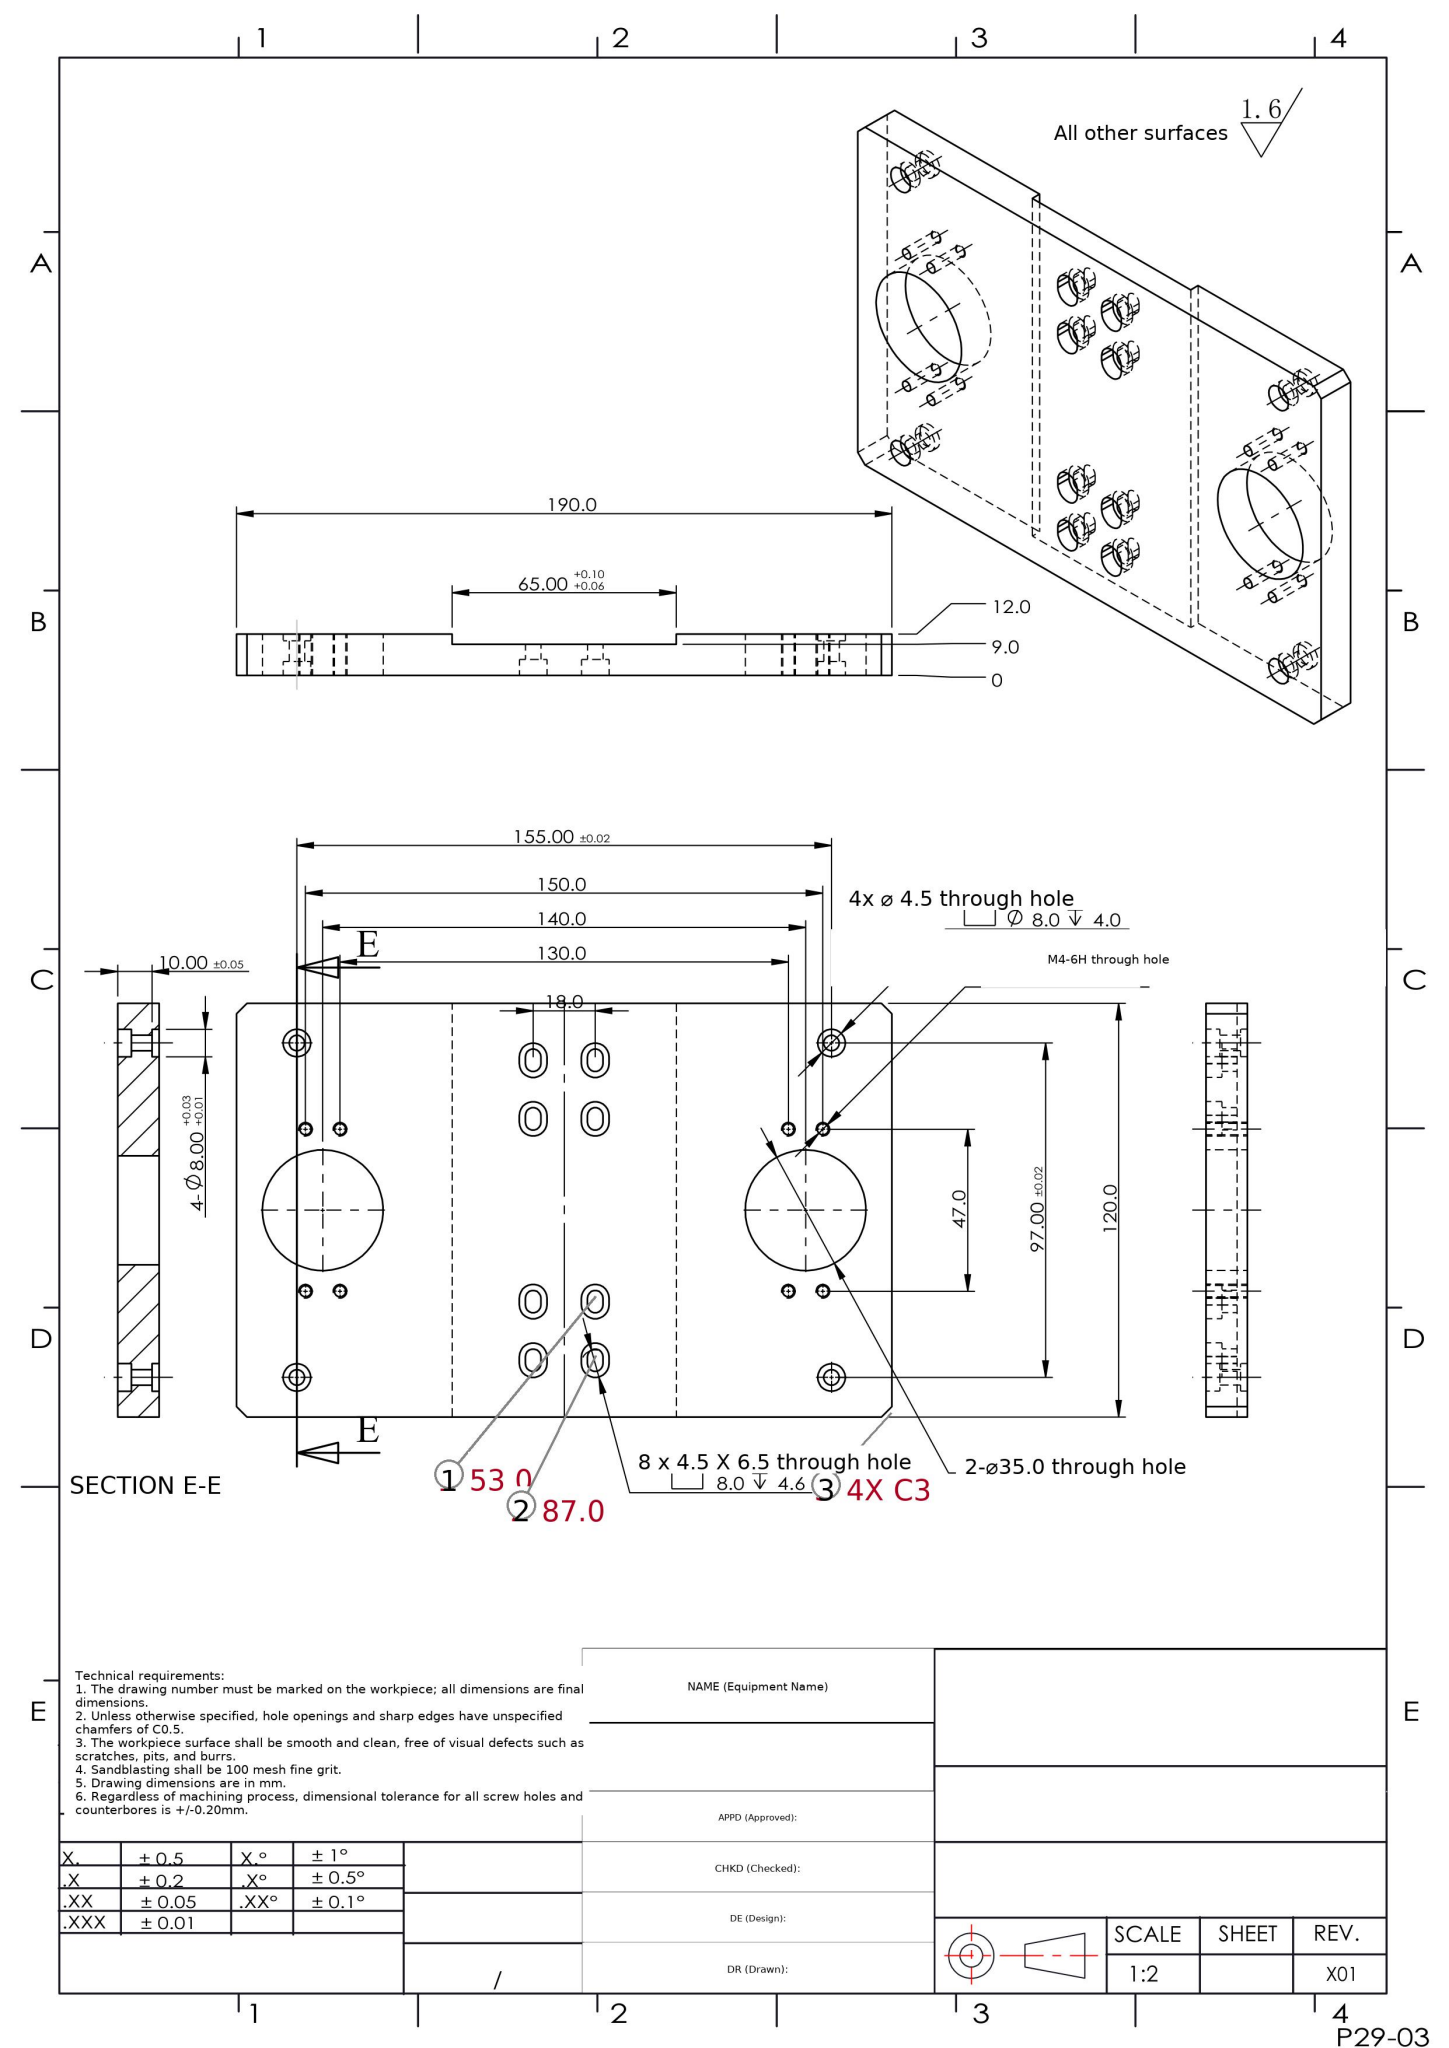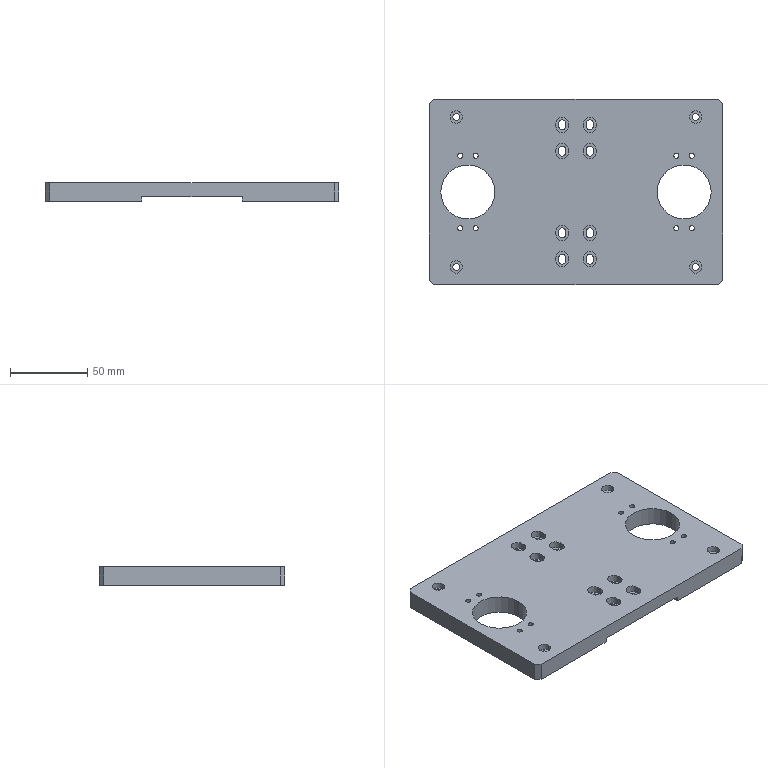Part | SolidWorks | mm | 1 solid | 138 faces | box 190 x 120 x 12 mm | volume 221169 mm3 | cylinder 76 | plane 62 | commonest cylinder face diameters 8 x32 4.5 x24 3.3 x16 35 x4